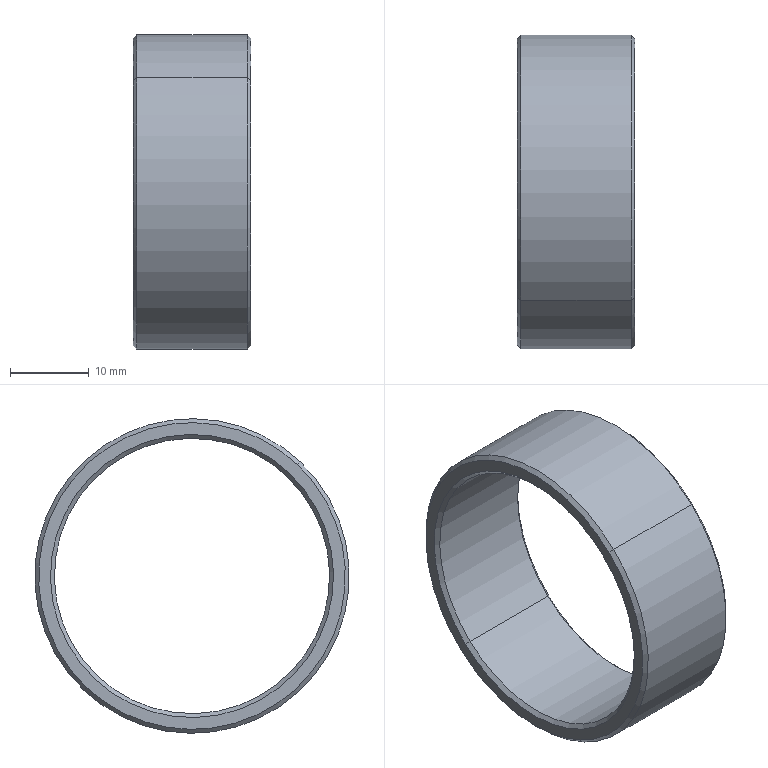Component | SolidWorks | 2-10-10WorkpieceAxisAssembly-1_2-10-4Bushing-1 | 1 solid | 14 faces | box 15 x 40 x 40 mm | volume 4359 mm3 | cone 8 | cylinder 4 | plane 2 | commonest cylinder face diameters 35 x2 40 x2
build123d program:
from build123d import *

# Parameters (mm, degrees)
SKETCH2_R      = 20
SKETCH2_R_2    = 17.5
EXTRUDE1_DEPTH = 15
CHAMFER1_SIZE  = 0.5


with BuildPart() as part:
    # Sketch2 → Extrude1 (new body)
    with BuildSketch(Plane(origin=(0, 0, 0), x_dir=(1, 0, 0), z_dir=(0, 1, 0))):
        with Locations(Location((0, 0, 0), (0, 0, 270))):
            Circle(SKETCH2_R)
        with Locations(Location((0, 0, 0), (0, 0, 270))):
            Circle(SKETCH2_R_2, mode=Mode.SUBTRACT)
    extrude(amount=EXTRUDE1_DEPTH)

    # Chamfer1
    chamfer1_edges = [part.edges().sort_by_distance(p)[0] for p in [
        (0, 0, -20),
        (0, 15, -20),
        (0, 0, -17.5),
        (0, 15, -17.5),
    ]]
    chamfer(chamfer1_edges, length=CHAMFER1_SIZE)


solid = part.part

# Placed as in the assembly
solid = solid.moved(Location((-475.809, -4.181, 0), (0, 0, 90)))
STEP:
#1=CARTESIAN_POINT('',(-19.304,-0.6388,0.4999));
#2=VERTEX_POINT('',#1);
#3=CARTESIAN_POINT('',(-19.304,0.3096,-0.4999));
#4=VERTEX_POINT('',#3);
#5=CARTESIAN_POINT('',(-19.304,-0.1646,-0.));
#6=DIRECTION('',(-1.,0.,-0.));
#7=DIRECTION('',(0.,0.6882,-0.7255));
#8=AXIS2_PLACEMENT_3D('',#5,#6,#7);
#9=CIRCLE('',#8,0.689);
#10=EDGE_CURVE('',#2,#4,#9,.T.);
#11=ORIENTED_EDGE('',*,*,#10,.F.);
#12=CARTESIAN_POINT('',(-19.323,-0.6523,0.5141));
#13=VERTEX_POINT('',#12);
#14=CARTESIAN_POINT('',(-19.304,-0.6388,0.4999));
#15=DIRECTION('',(-0.7071,-0.4866,0.513));
#16=VECTOR('',#15,39.37);
#17=LINE('',#14,#16);
#18=EDGE_CURVE('',#2,#13,#17,.T.);
#19=ORIENTED_EDGE('',*,*,#18,.T.);
#20=CARTESIAN_POINT('',(-19.323,0.3231,-0.5141));
#21=VERTEX_POINT('',#20);
#22=CARTESIAN_POINT('',(-19.323,-0.1646,-0.));
#23=DIRECTION('',(1.,-0.,0.));
#24=DIRECTION('',(0.,0.6882,-0.7255));
#25=AXIS2_PLACEMENT_3D('',#22,#23,#24);
#26=CIRCLE('',#25,0.7087);
#27=EDGE_CURVE('',#21,#13,#26,.T.);
#28=ORIENTED_EDGE('',*,*,#27,.F.);
#29=CARTESIAN_POINT('',(-19.304,0.3096,-0.4999));
#30=DIRECTION('',(-0.7071,0.4866,-0.513));
#31=VECTOR('',#30,39.37);
#32=LINE('',#29,#31);
#33=EDGE_CURVE('',#4,#21,#32,.T.);
#34=ORIENTED_EDGE('',*,*,#33,.F.);
#35=EDGE_LOOP('',(#11,#19,#28,#34));
#36=FACE_OUTER_BOUND('',#35,.T.);
#37=CARTESIAN_POINT('',(-19.304,-0.1646,-0.));
#38=DIRECTION('',(-1.,0.,-0.));
#39=DIRECTION('',(0.,0.6882,-0.7255));
#40=AXIS2_PLACEMENT_3D('',#37,#38,#39);
#41=CONICAL_SURFACE('',#40,0.689,0.7854);
#42=ADVANCED_FACE('',(#36),#41,.F.);
#43=CARTESIAN_POINT('',(-19.323,0.3637,-0.557));
#44=VERTEX_POINT('',#43);
#45=CARTESIAN_POINT('',(-19.323,-0.693,0.557));
#46=VERTEX_POINT('',#45);
#47=CARTESIAN_POINT('',(-19.323,-0.1646,-0.));
#48=DIRECTION('',(-1.,0.,-0.));
#49=DIRECTION('',(0.,0.6882,-0.7255));
#50=AXIS2_PLACEMENT_3D('',#47,#48,#49);
#51=CIRCLE('',#50,0.7677);
#52=EDGE_CURVE('',#44,#46,#51,.T.);
#53=ORIENTED_EDGE('',*,*,#52,.F.);
#54=CARTESIAN_POINT('',(-19.304,0.3773,-0.5713));
#55=VERTEX_POINT('',#54);
#56=CARTESIAN_POINT('',(-19.323,0.3637,-0.557));
#57=DIRECTION('',(0.7071,0.4866,-0.513));
#58=VECTOR('',#57,39.37);
#59=LINE('',#56,#58);
#60=EDGE_CURVE('',#44,#55,#59,.T.);
#61=ORIENTED_EDGE('',*,*,#60,.T.);
#62=CARTESIAN_POINT('',(-19.304,-0.7065,0.5713));
#63=VERTEX_POINT('',#62);
#64=CARTESIAN_POINT('',(-19.304,-0.1646,-0.));
#65=DIRECTION('',(1.,-0.,0.));
#66=DIRECTION('',(0.,0.6882,-0.7255));
#67=AXIS2_PLACEMENT_3D('',#64,#65,#66);
#68=CIRCLE('',#67,0.7874);
#69=EDGE_CURVE('',#63,#55,#68,.T.);
#70=ORIENTED_EDGE('',*,*,#69,.F.);
#71=CARTESIAN_POINT('',(-19.323,-0.693,0.557));
#72=DIRECTION('',(0.7071,-0.4866,0.513));
#73=VECTOR('',#72,39.37);
#74=LINE('',#71,#73);
#75=EDGE_CURVE('',#46,#63,#74,.T.);
#76=ORIENTED_EDGE('',*,*,#75,.F.);
#77=EDGE_LOOP('',(#53,#61,#70,#76));
#78=FACE_OUTER_BOUND('',#77,.T.);
#79=CARTESIAN_POINT('',(-19.323,-0.1646,-0.));
#80=DIRECTION('',(1.,-0.,0.));
#81=DIRECTION('',(0.,-0.6882,0.7255));
#82=AXIS2_PLACEMENT_3D('',#79,#80,#81);
#83=CONICAL_SURFACE('',#82,0.7677,0.7854);
#84=ADVANCED_FACE('',(#78),#83,.T.);
#85=CARTESIAN_POINT('',(-18.733,-0.693,0.557));
#86=VERTEX_POINT('',#85);
#87=CARTESIAN_POINT('',(-18.733,0.3637,-0.557));
#88=VERTEX_POINT('',#87);
#89=CARTESIAN_POINT('',(-18.733,-0.1646,-0.));
#90=DIRECTION('',(1.,-0.,0.));
#91=DIRECTION('',(0.,0.6882,-0.7255));
#92=AXIS2_PLACEMENT_3D('',#89,#90,#91);
#93=CIRCLE('',#92,0.7677);
#94=EDGE_CURVE('',#86,#88,#93,.T.);
#95=ORIENTED_EDGE('',*,*,#94,.F.);
#96=CARTESIAN_POINT('',(-18.752,-0.7065,0.5713));
#97=VERTEX_POINT('',#96);
#98=CARTESIAN_POINT('',(-18.752,-0.7065,0.5713));
#99=DIRECTION('',(-0.7071,-0.4866,0.513));
#100=VECTOR('',#99,39.37);
#101=LINE('',#98,#100);
#102=EDGE_CURVE('',#86,#97,#101,.T.);
#103=ORIENTED_EDGE('',*,*,#102,.T.);
#104=CARTESIAN_POINT('',(-18.752,0.3773,-0.5713));
#105=VERTEX_POINT('',#104);
#106=CARTESIAN_POINT('',(-18.752,-0.1646,-0.));
#107=DIRECTION('',(-1.,0.,-0.));
#108=DIRECTION('',(0.,0.6882,-0.7255));
#109=AXIS2_PLACEMENT_3D('',#106,#107,#108);
#110=CIRCLE('',#109,0.7874);
#111=EDGE_CURVE('',#105,#97,#110,.T.);
#112=ORIENTED_EDGE('',*,*,#111,.F.);
#113=CARTESIAN_POINT('',(-18.752,0.3773,-0.5713));
#114=DIRECTION('',(-0.7071,0.4866,-0.513));
#115=VECTOR('',#114,39.37);
#116=LINE('',#113,#115);
#117=EDGE_CURVE('',#88,#105,#116,.T.);
#118=ORIENTED_EDGE('',*,*,#117,.F.);
#119=EDGE_LOOP('',(#95,#103,#112,#118));
#120=FACE_OUTER_BOUND('',#119,.T.);
#121=CARTESIAN_POINT('',(-18.752,-0.1646,-0.));
#122=DIRECTION('',(-1.,0.,-0.));
#123=DIRECTION('',(0.,0.6882,-0.7255));
#124=AXIS2_PLACEMENT_3D('',#121,#122,#123);
#125=CONICAL_SURFACE('',#124,0.7874,0.7854);
#126=ADVANCED_FACE('',(#120),#125,.T.);
#127=CARTESIAN_POINT('',(-18.752,0.3096,-0.4999));
#128=VERTEX_POINT('',#127);
#129=CARTESIAN_POINT('',(-18.752,-0.6388,0.4999));
#130=VERTEX_POINT('',#129);
#131=CARTESIAN_POINT('',(-18.752,-0.1646,-0.));
#132=DIRECTION('',(1.,-0.,0.));
#133=DIRECTION('',(0.,0.6882,-0.7255));
#134=AXIS2_PLACEMENT_3D('',#131,#132,#133);
#135=CIRCLE('',#134,0.689);
#136=EDGE_CURVE('',#128,#130,#135,.T.);
#137=ORIENTED_EDGE('',*,*,#136,.F.);
#138=CARTESIAN_POINT('',(-18.733,0.3231,-0.5141));
#139=VERTEX_POINT('',#138);
#140=CARTESIAN_POINT('',(-18.733,0.3231,-0.5141));
#141=DIRECTION('',(0.7071,0.4866,-0.513));
#142=VECTOR('',#141,39.37);
#143=LINE('',#140,#142);
#144=EDGE_CURVE('',#128,#139,#143,.T.);
#145=ORIENTED_EDGE('',*,*,#144,.T.);
#146=CARTESIAN_POINT('',(-18.733,-0.6523,0.5141));
#147=VERTEX_POINT('',#146);
#148=CARTESIAN_POINT('',(-18.733,-0.1646,-0.));
#149=DIRECTION('',(-1.,0.,-0.));
#150=DIRECTION('',(0.,0.6882,-0.7255));
#151=AXIS2_PLACEMENT_3D('',#148,#149,#150);
#152=CIRCLE('',#151,0.7087);
#153=EDGE_CURVE('',#147,#139,#152,.T.);
#154=ORIENTED_EDGE('',*,*,#153,.F.);
#155=CARTESIAN_POINT('',(-18.733,-0.6523,0.5141));
#156=DIRECTION('',(0.7071,-0.4866,0.513));
#157=VECTOR('',#156,39.37);
#158=LINE('',#155,#157);
#159=EDGE_CURVE('',#130,#147,#158,.T.);
#160=ORIENTED_EDGE('',*,*,#159,.F.);
#161=EDGE_LOOP('',(#137,#145,#154,#160));
#162=FACE_OUTER_BOUND('',#161,.T.);
#163=CARTESIAN_POINT('',(-18.733,-0.1646,-0.));
#164=DIRECTION('',(1.,-0.,0.));
#165=DIRECTION('',(0.,-0.6882,0.7255));
#166=AXIS2_PLACEMENT_3D('',#163,#164,#165);
#167=CONICAL_SURFACE('',#166,0.7087,0.7854);
#168=ADVANCED_FACE('',(#162),#167,.F.);
#169=ORIENTED_EDGE('',*,*,#10,.T.);
#170=CARTESIAN_POINT('',(-19.323,0.3096,-0.4999));
#171=DIRECTION('',(1.,-0.,0.));
#172=VECTOR('',#171,39.37);
#173=LINE('',#170,#172);
#174=EDGE_CURVE('',#4,#128,#173,.T.);
#175=ORIENTED_EDGE('',*,*,#174,.T.);
#176=ORIENTED_EDGE('',*,*,#136,.T.);
#177=CARTESIAN_POINT('',(-19.323,-0.6388,0.4999));
#178=DIRECTION('',(1.,-0.,0.));
#179=VECTOR('',#178,39.37);
#180=LINE('',#177,#179);
#181=EDGE_CURVE('',#2,#130,#180,.T.);
#182=ORIENTED_EDGE('',*,*,#181,.F.);
#183=EDGE_LOOP('',(#169,#175,#176,#182));
#184=FACE_OUTER_BOUND('',#183,.T.);
#185=CARTESIAN_POINT('',(-19.323,-0.1646,-0.));
#186=DIRECTION('',(1.,-0.,0.));
#187=DIRECTION('',(0.,-0.6882,0.7255));
#188=AXIS2_PLACEMENT_3D('',#185,#186,#187);
#189=CYLINDRICAL_SURFACE('',#188,0.689);
#190=ADVANCED_FACE('',(#184),#189,.F.);
#191=ORIENTED_EDGE('',*,*,#69,.T.);
#192=CARTESIAN_POINT('',(-19.323,0.3773,-0.5713));
#193=DIRECTION('',(1.,-0.,0.));
#194=VECTOR('',#193,39.37);
#195=LINE('',#192,#194);
#196=EDGE_CURVE('',#55,#105,#195,.T.);
#197=ORIENTED_EDGE('',*,*,#196,.T.);
#198=ORIENTED_EDGE('',*,*,#111,.T.);
#199=CARTESIAN_POINT('',(-19.323,-0.7065,0.5713));
#200=DIRECTION('',(1.,-0.,0.));
#201=VECTOR('',#200,39.37);
#202=LINE('',#199,#201);
#203=EDGE_CURVE('',#63,#97,#202,.T.);
#204=ORIENTED_EDGE('',*,*,#203,.F.);
#205=EDGE_LOOP('',(#191,#197,#198,#204));
#206=FACE_OUTER_BOUND('',#205,.T.);
#207=CARTESIAN_POINT('',(-19.323,-0.1646,-0.));
#208=DIRECTION('',(1.,-0.,0.));
#209=DIRECTION('',(0.,-0.6882,0.7255));
#210=AXIS2_PLACEMENT_3D('',#207,#208,#209);
#211=CYLINDRICAL_SURFACE('',#210,0.7874);
#212=ADVANCED_FACE('',(#206),#211,.T.);
#213=CARTESIAN_POINT('',(-19.323,-0.1646,-0.));
#214=DIRECTION('',(-1.,0.,-0.));
#215=DIRECTION('',(0.,0.6882,-0.7255));
#216=AXIS2_PLACEMENT_3D('',#213,#214,#215);
#217=CIRCLE('',#216,0.7677);
#218=EDGE_CURVE('',#46,#44,#217,.T.);
#219=ORIENTED_EDGE('',*,*,#218,.T.);
#220=ORIENTED_EDGE('',*,*,#52,.T.);
#221=EDGE_LOOP('',(#219,#220));
#222=FACE_OUTER_BOUND('',#221,.T.);
#223=ORIENTED_EDGE('',*,*,#27,.T.);
#224=CARTESIAN_POINT('',(-19.323,-0.1646,-0.));
#225=DIRECTION('',(1.,-0.,0.));
#226=DIRECTION('',(0.,0.6882,-0.7255));
#227=AXIS2_PLACEMENT_3D('',#224,#225,#226);
#228=CIRCLE('',#227,0.7087);
#229=EDGE_CURVE('',#13,#21,#228,.T.);
#230=ORIENTED_EDGE('',*,*,#229,.T.);
#231=EDGE_LOOP('',(#223,#230));
#232=FACE_BOUND('',#231,.T.);
#233=CARTESIAN_POINT('',(-19.323,-0.1646,-0.));
#234=DIRECTION('',(-1.,0.,-0.));
#235=DIRECTION('',(0.,0.6882,-0.7255));
#236=AXIS2_PLACEMENT_3D('',#233,#234,#235);
#237=PLANE('',#236);
#238=ADVANCED_FACE('',(#222,#232),#237,.T.);
#239=ORIENTED_EDGE('',*,*,#153,.T.);
#240=CARTESIAN_POINT('',(-18.733,-0.1646,-0.));
#241=DIRECTION('',(-1.,0.,-0.));
#242=DIRECTION('',(0.,0.6882,-0.7255));
#243=AXIS2_PLACEMENT_3D('',#240,#241,#242);
#244=CIRCLE('',#243,0.7087);
#245=EDGE_CURVE('',#139,#147,#244,.T.);
#246=ORIENTED_EDGE('',*,*,#245,.T.);
#247=EDGE_LOOP('',(#239,#246));
#248=FACE_BOUND('',#247,.T.);
#249=CARTESIAN_POINT('',(-18.733,-0.1646,-0.));
#250=DIRECTION('',(1.,-0.,0.));
#251=DIRECTION('',(0.,0.6882,-0.7255));
#252=AXIS2_PLACEMENT_3D('',#249,#250,#251);
#253=CIRCLE('',#252,0.7677);
#254=EDGE_CURVE('',#88,#86,#253,.T.);
#255=ORIENTED_EDGE('',*,*,#254,.T.);
#256=ORIENTED_EDGE('',*,*,#94,.T.);
#257=EDGE_LOOP('',(#255,#256));
#258=FACE_OUTER_BOUND('',#257,.T.);
#259=CARTESIAN_POINT('',(-18.733,-0.1646,-0.));
#260=DIRECTION('',(-1.,0.,-0.));
#261=DIRECTION('',(0.,0.6882,-0.7255));
#262=AXIS2_PLACEMENT_3D('',#259,#260,#261);
#263=PLANE('',#262);
#264=ADVANCED_FACE('',(#248,#258),#263,.F.);
#265=ORIENTED_EDGE('',*,*,#196,.F.);
#266=CARTESIAN_POINT('',(-19.304,-0.1646,-0.));
#267=DIRECTION('',(1.,-0.,0.));
#268=DIRECTION('',(0.,0.6882,-0.7255));
#269=AXIS2_PLACEMENT_3D('',#266,#267,#268);
#270=CIRCLE('',#269,0.7874);
#271=EDGE_CURVE('',#55,#63,#270,.T.);
#272=ORIENTED_EDGE('',*,*,#271,.T.);
#273=ORIENTED_EDGE('',*,*,#203,.T.);
#274=CARTESIAN_POINT('',(-18.752,-0.1646,-0.));
#275=DIRECTION('',(-1.,0.,-0.));
#276=DIRECTION('',(0.,0.6882,-0.7255));
#277=AXIS2_PLACEMENT_3D('',#274,#275,#276);
#278=CIRCLE('',#277,0.7874);
#279=EDGE_CURVE('',#97,#105,#278,.T.);
#280=ORIENTED_EDGE('',*,*,#279,.T.);
#281=EDGE_LOOP('',(#265,#272,#273,#280));
#282=FACE_OUTER_BOUND('',#281,.T.);
#283=CARTESIAN_POINT('',(-19.323,-0.1646,-0.));
#284=DIRECTION('',(1.,-0.,0.));
#285=DIRECTION('',(0.,-0.6882,0.7255));
#286=AXIS2_PLACEMENT_3D('',#283,#284,#285);
#287=CYLINDRICAL_SURFACE('',#286,0.7874);
#288=ADVANCED_FACE('',(#282),#287,.T.);
#289=ORIENTED_EDGE('',*,*,#174,.F.);
#290=CARTESIAN_POINT('',(-19.304,-0.1646,-0.));
#291=DIRECTION('',(-1.,0.,-0.));
#292=DIRECTION('',(0.,0.6882,-0.7255));
#293=AXIS2_PLACEMENT_3D('',#290,#291,#292);
#294=CIRCLE('',#293,0.689);
#295=EDGE_CURVE('',#4,#2,#294,.T.);
#296=ORIENTED_EDGE('',*,*,#295,.T.);
#297=ORIENTED_EDGE('',*,*,#181,.T.);
#298=CARTESIAN_POINT('',(-18.752,-0.1646,-0.));
#299=DIRECTION('',(1.,-0.,0.));
#300=DIRECTION('',(0.,0.6882,-0.7255));
#301=AXIS2_PLACEMENT_3D('',#298,#299,#300);
#302=CIRCLE('',#301,0.689);
#303=EDGE_CURVE('',#130,#128,#302,.T.);
#304=ORIENTED_EDGE('',*,*,#303,.T.);
#305=EDGE_LOOP('',(#289,#296,#297,#304));
#306=FACE_OUTER_BOUND('',#305,.T.);
#307=CARTESIAN_POINT('',(-19.323,-0.1646,-0.));
#308=DIRECTION('',(1.,-0.,0.));
#309=DIRECTION('',(0.,-0.6882,0.7255));
#310=AXIS2_PLACEMENT_3D('',#307,#308,#309);
#311=CYLINDRICAL_SURFACE('',#310,0.689);
#312=ADVANCED_FACE('',(#306),#311,.F.);
#313=ORIENTED_EDGE('',*,*,#144,.F.);
#314=ORIENTED_EDGE('',*,*,#303,.F.);
#315=ORIENTED_EDGE('',*,*,#159,.T.);
#316=ORIENTED_EDGE('',*,*,#245,.F.);
#317=EDGE_LOOP('',(#313,#314,#315,#316));
#318=FACE_OUTER_BOUND('',#317,.T.);
#319=CARTESIAN_POINT('',(-18.733,-0.1646,-0.));
#320=DIRECTION('',(1.,-0.,0.));
#321=DIRECTION('',(0.,-0.6882,0.7255));
#322=AXIS2_PLACEMENT_3D('',#319,#320,#321);
#323=CONICAL_SURFACE('',#322,0.7087,0.7854);
#324=ADVANCED_FACE('',(#318),#323,.F.);
#325=ORIENTED_EDGE('',*,*,#102,.F.);
#326=ORIENTED_EDGE('',*,*,#254,.F.);
#327=ORIENTED_EDGE('',*,*,#117,.T.);
#328=ORIENTED_EDGE('',*,*,#279,.F.);
#329=EDGE_LOOP('',(#325,#326,#327,#328));
#330=FACE_OUTER_BOUND('',#329,.T.);
#331=CARTESIAN_POINT('',(-18.752,-0.1646,-0.));
#332=DIRECTION('',(-1.,0.,-0.));
#333=DIRECTION('',(0.,0.6882,-0.7255));
#334=AXIS2_PLACEMENT_3D('',#331,#332,#333);
#335=CONICAL_SURFACE('',#334,0.7874,0.7854);
#336=ADVANCED_FACE('',(#330),#335,.T.);
#337=ORIENTED_EDGE('',*,*,#60,.F.);
#338=ORIENTED_EDGE('',*,*,#218,.F.);
#339=ORIENTED_EDGE('',*,*,#75,.T.);
#340=ORIENTED_EDGE('',*,*,#271,.F.);
#341=EDGE_LOOP('',(#337,#338,#339,#340));
#342=FACE_OUTER_BOUND('',#341,.T.);
#343=CARTESIAN_POINT('',(-19.323,-0.1646,-0.));
#344=DIRECTION('',(1.,-0.,0.));
#345=DIRECTION('',(0.,-0.6882,0.7255));
#346=AXIS2_PLACEMENT_3D('',#343,#344,#345);
#347=CONICAL_SURFACE('',#346,0.7677,0.7854);
#348=ADVANCED_FACE('',(#342),#347,.T.);
#349=ORIENTED_EDGE('',*,*,#18,.F.);
#350=ORIENTED_EDGE('',*,*,#295,.F.);
#351=ORIENTED_EDGE('',*,*,#33,.T.);
#352=ORIENTED_EDGE('',*,*,#229,.F.);
#353=EDGE_LOOP('',(#349,#350,#351,#352));
#354=FACE_OUTER_BOUND('',#353,.T.);
#355=CARTESIAN_POINT('',(-19.304,-0.1646,-0.));
#356=DIRECTION('',(-1.,0.,-0.));
#357=DIRECTION('',(0.,0.6882,-0.7255));
#358=AXIS2_PLACEMENT_3D('',#355,#356,#357);
#359=CONICAL_SURFACE('',#358,0.689,0.7854);
#360=ADVANCED_FACE('',(#354),#359,.F.);
#361=CLOSED_SHELL('',(#42,#84,#126,#168,#190,#212,#238,#264,#288,#312,#324,#336,#348,#360));
#362=MANIFOLD_SOLID_BREP('',#361);
#363=CARTESIAN_POINT('',(0.,0.,0.));
#364=DIRECTION('',(0.,0.,1.));
#365=DIRECTION('',(1.,0.,0.));
#366=AXIS2_PLACEMENT_3D('',#363,#364,#365);
#367=(LENGTH_UNIT()NAMED_UNIT(*)SI_UNIT($,.METRE.));
#368=LENGTH_MEASURE_WITH_UNIT(LENGTH_MEASURE(0.0254),#367);
#369=DIMENSIONAL_EXPONENTS(1.,0.,0.,0.,0.,0.,0.);
#370=(CONVERSION_BASED_UNIT('',#368)LENGTH_UNIT()NAMED_UNIT(#369));
#371=UNCERTAINTY_MEASURE_WITH_UNIT(LENGTH_MEASURE(0.00001),#370,'','');
#372=(NAMED_UNIT(*)PLANE_ANGLE_UNIT()SI_UNIT($,.RADIAN.));
#373=(NAMED_UNIT(*)SI_UNIT($,.STERADIAN.)SOLID_ANGLE_UNIT());
#374=(GEOMETRIC_REPRESENTATION_CONTEXT(3)GLOBAL_UNCERTAINTY_ASSIGNED_CONTEXT((#371))GLOBAL_UNIT_ASSIGNED_CONTEXT((#370,#372,#373))REPRESENTATION_CONTEXT('',''));
#375=ADVANCED_BREP_SHAPE_REPRESENTATION('',(#362,#366),#374);
#376=COLOUR_RGB('',0.7922,0.8196,0.9333);
#377=FILL_AREA_STYLE_COLOUR('',#376);
#378=FILL_AREA_STYLE('',(#377));
#379=SURFACE_STYLE_FILL_AREA(#378);
#380=SURFACE_SIDE_STYLE('',(#379));
#381=SURFACE_STYLE_USAGE(.BOTH.,#380);
#382=PRESENTATION_STYLE_ASSIGNMENT((#381));
#383=STYLED_ITEM('',(#382),#362);
#384=PRESENTATION_LAYER_ASSIGNMENT('','',(#383));
#385=(LENGTH_UNIT()NAMED_UNIT(*)SI_UNIT($,.METRE.));
#386=LENGTH_MEASURE_WITH_UNIT(LENGTH_MEASURE(0.0254),#385);
#387=DIMENSIONAL_EXPONENTS(1.,0.,0.,0.,0.,0.,0.);
#388=(CONVERSION_BASED_UNIT('',#386)LENGTH_UNIT()NAMED_UNIT(#387));
#389=UNCERTAINTY_MEASURE_WITH_UNIT(LENGTH_MEASURE(0.00001),#388,'','');
#390=(NAMED_UNIT(*)PLANE_ANGLE_UNIT()SI_UNIT($,.RADIAN.));
#391=(NAMED_UNIT(*)SI_UNIT($,.STERADIAN.)SOLID_ANGLE_UNIT());
#392=(GEOMETRIC_REPRESENTATION_CONTEXT(3)GLOBAL_UNCERTAINTY_ASSIGNED_CONTEXT((#389))GLOBAL_UNIT_ASSIGNED_CONTEXT((#388,#390,#391))REPRESENTATION_CONTEXT('',''));
#393=MECHANICAL_DESIGN_GEOMETRIC_PRESENTATION_REPRESENTATION('',(#383),#392);